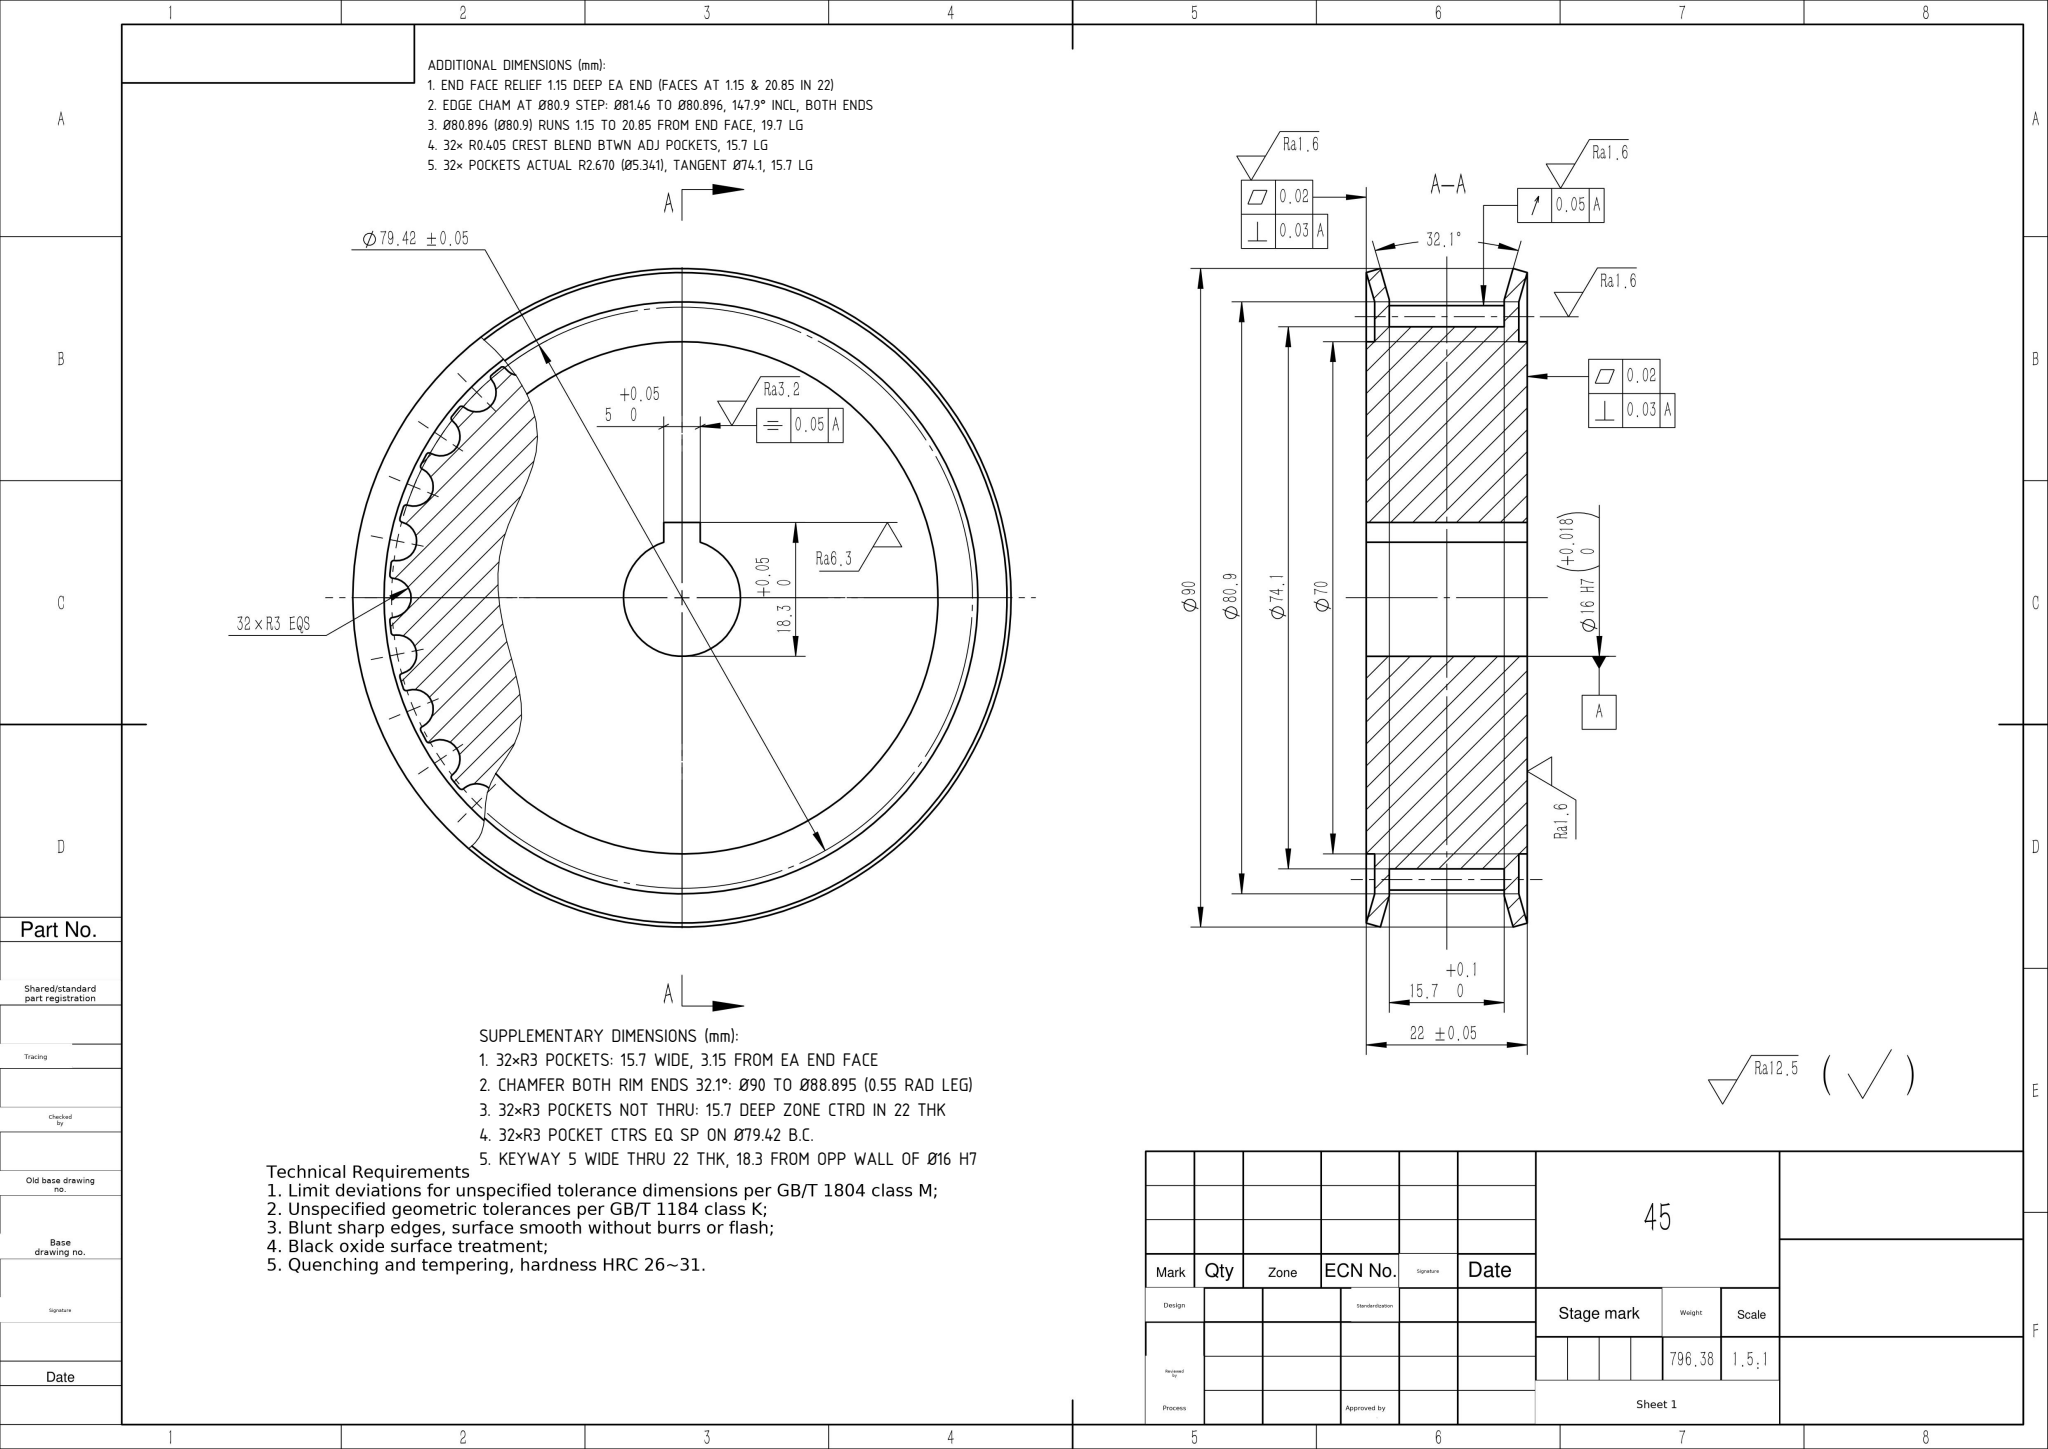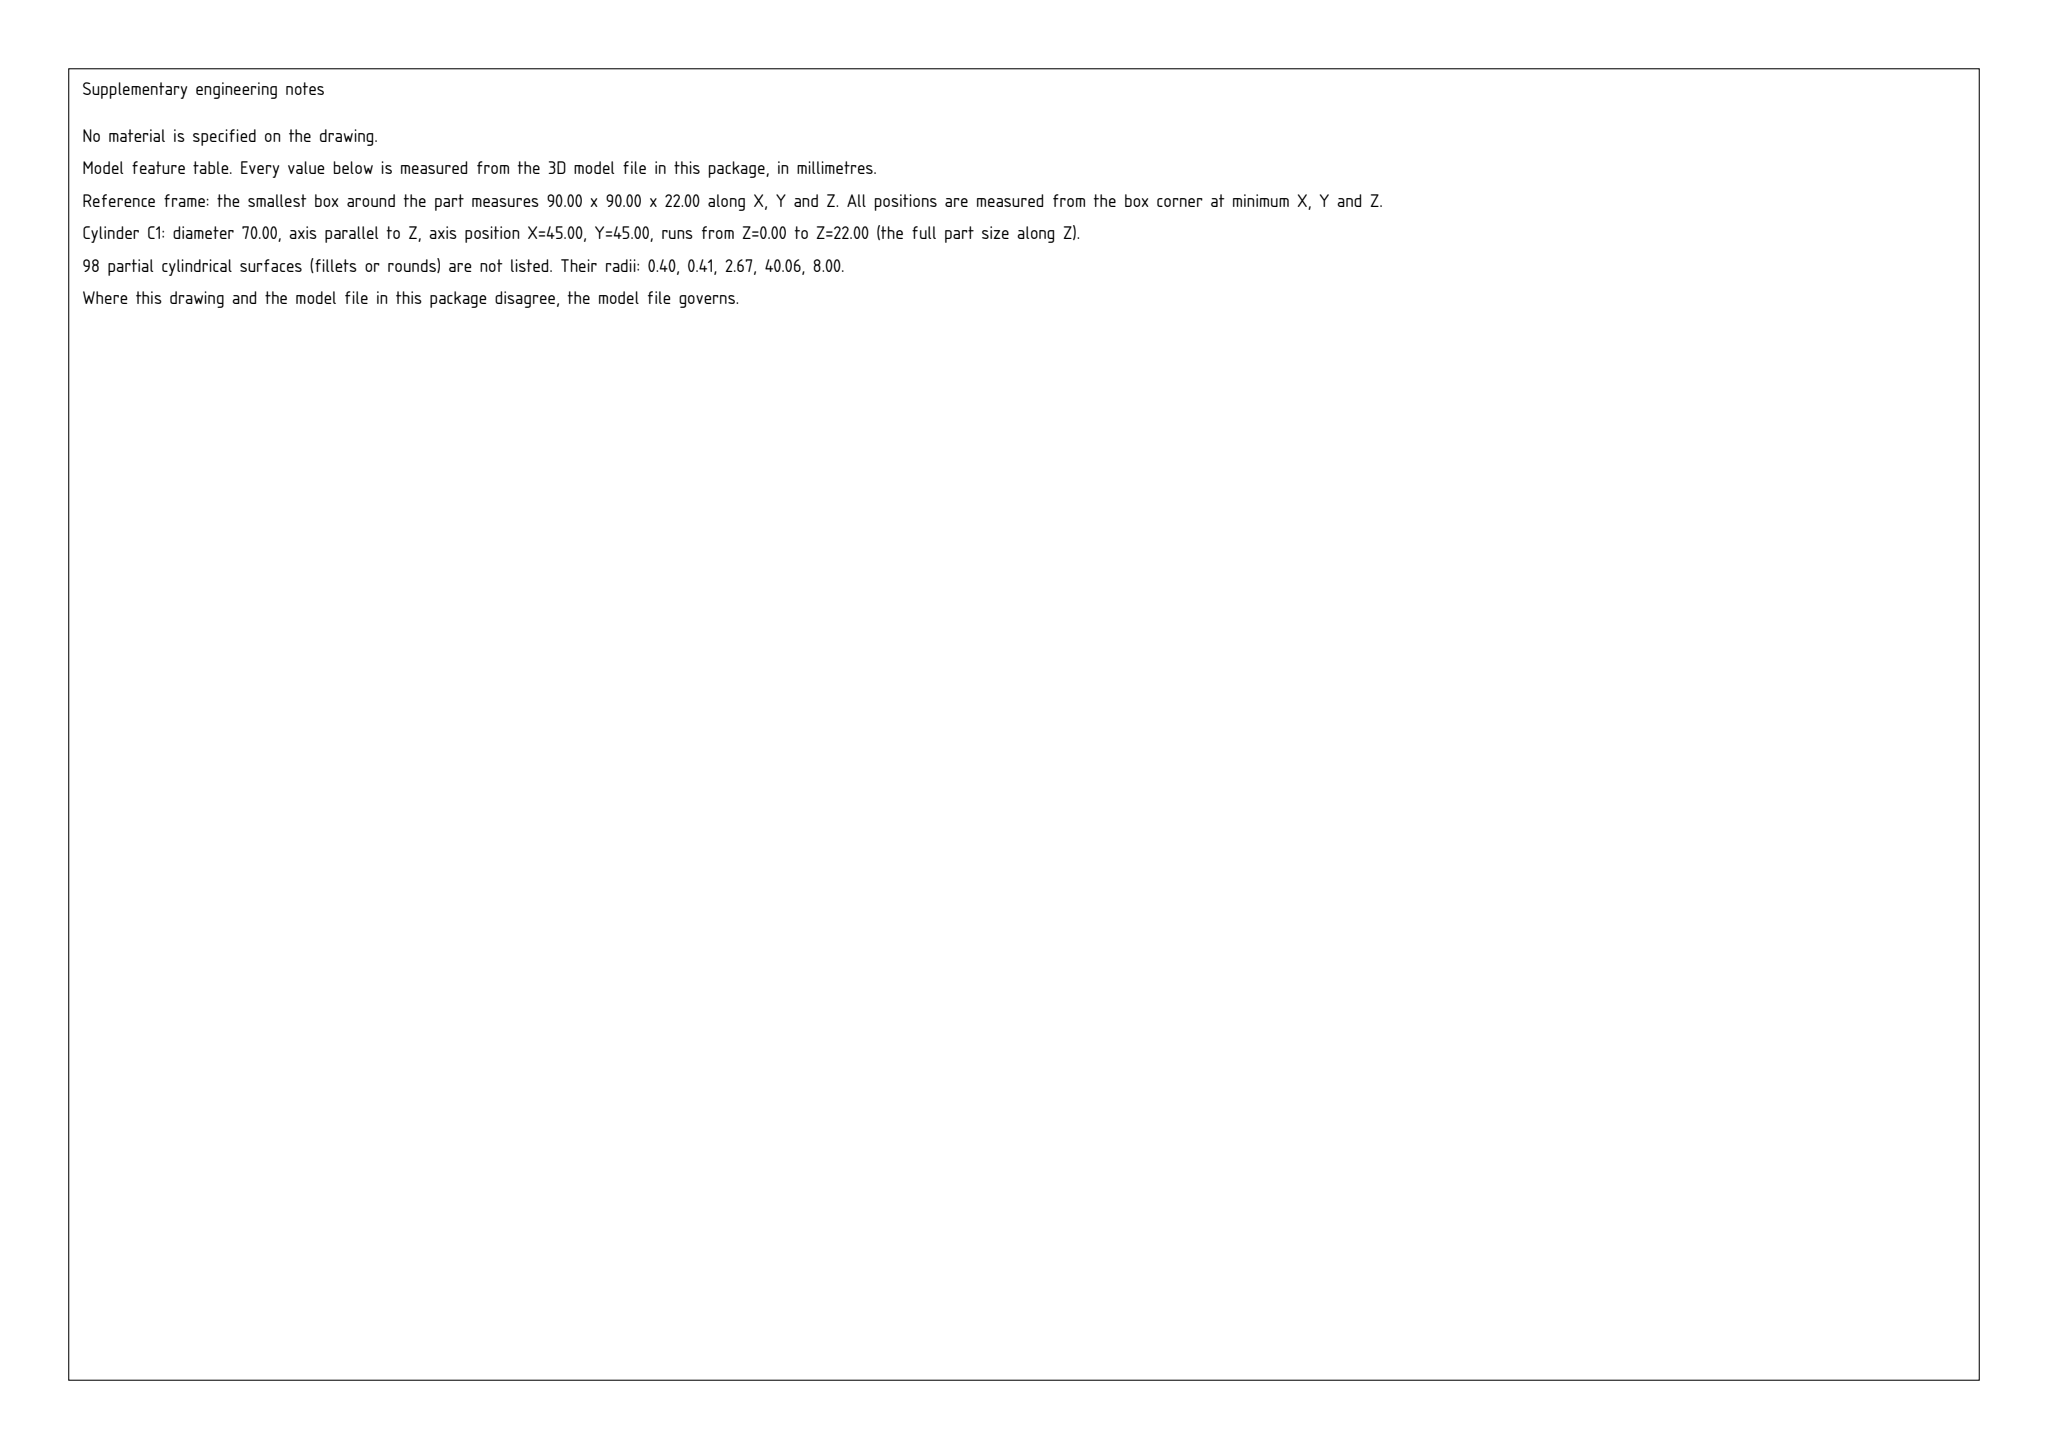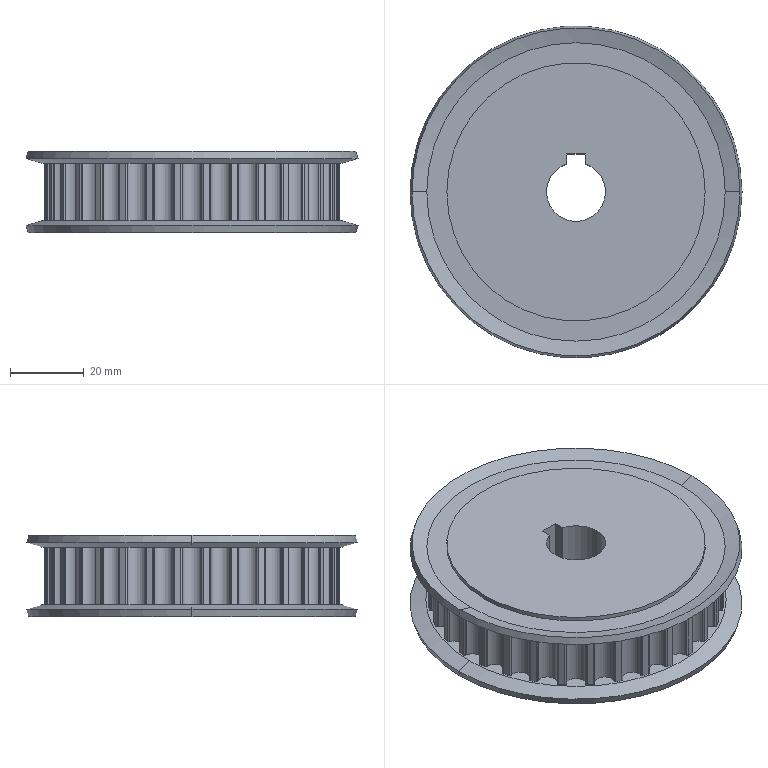Part | SolidWorks | mm | 1 solid | 251 faces | box 90 x 90 x 22 mm | volume 102100 mm3 | cylinder 166 | plane 73 | cone 12 | commonest cylinder face diameters 0.81 x80 5.341 x47 80.12 x32 70 x4 16 x3